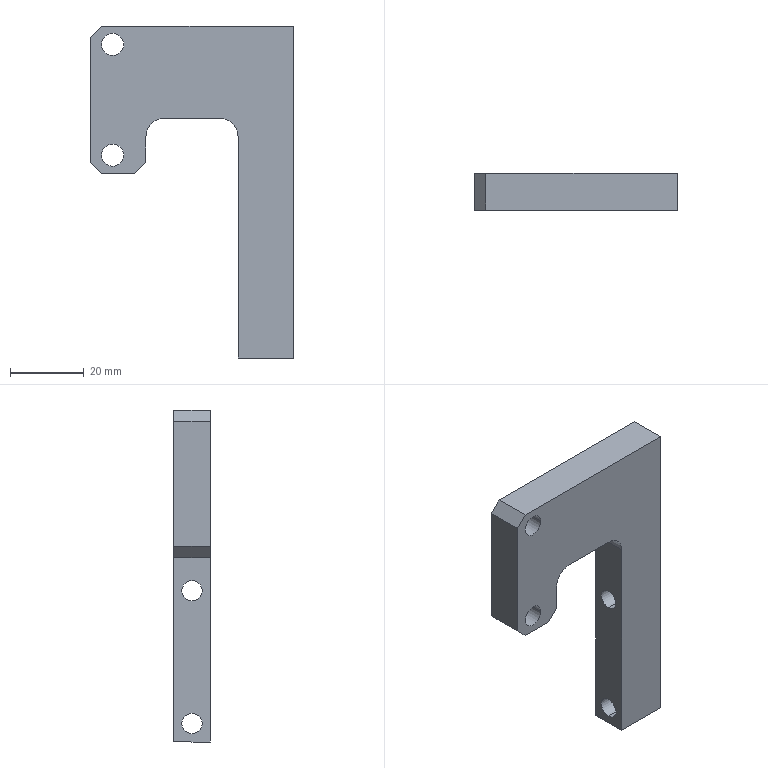Component | SolidWorks | JL001-05-01-011-1 | 1 solid | 23 faces | box 55 x 10 x 90 mm | volume 24444 mm3 | plane 13 | cylinder 10 | commonest cylinder face diameters 6 x4 5.5 x4 10 x2
build123d program:
from build123d import *

# Parameters (mm, degrees)
SKETCH1_W                  = 90
SKETCH1_H                  = 55
BOSS_EXTRUDE1_DEPTH        = 5
SKETCH2_W                  = 50
SKETCH2_H                  = 40
CUT_EXTRUDE1_DEPTH         = 54.677
SKETCH7_W                  = 15
SKETCH7_H                  = 25
CUT_EXTRUDE2_DEPTH         = 10
FILLET1_R                  = 5
F_5_5_5_5_DIAMETER_HOLE1_D = 5.5
M6_TAPPED_HOLE1_D          = 6
CHAMFER1_SIZE              = 3


with BuildPart() as part:
    # Sketch1 → Boss-Extrude1 (new, symmetric)
    with BuildSketch(Plane(origin=(0, 0, 0), x_dir=(1, 0, 0), z_dir=(0, 1, 0))):
        Rectangle(SKETCH1_W, SKETCH1_H)
    extrude(amount=BOSS_EXTRUDE1_DEPTH, both=True)

    # Sketch2 → Cut-Extrude1 (cut, through all)
    with BuildSketch(Plane(origin=(0, 5, 0), x_dir=(1, 0, 0), z_dir=(0, 1, 0))):
        with Locations((-20, -7.5)):
            Rectangle(SKETCH2_W, SKETCH2_H)
    extrude(amount=-CUT_EXTRUDE1_DEPTH, mode=Mode.SUBTRACT)

    # Sketch7 → Cut-Extrude2 (cut)
    with BuildSketch(Plane(origin=(0, 5, 0), x_dir=(1, 0, 0), z_dir=(0, 1, 0))):
        with Locations((12.5, 0)):
            Rectangle(SKETCH7_W, SKETCH7_H)
    extrude(amount=-CUT_EXTRUDE2_DEPTH, mode=Mode.SUBTRACT)

    # Fillet1
    fillet1_edges = [part.edges().sort_by_distance(p)[0] for p in [
        (20, 0, -12.5),
        (20, 0, 12.5),
    ]]
    fillet(fillet1_edges, radius=FILLET1_R)

    # 5.5 _5.5_ Diameter Hole1 (through all)
    with Locations(Plane.XY.offset(-12.5)):
        with Locations((-40, 0), (-4, 0)):
            Hole(F_5_5_5_5_DIAMETER_HOLE1_D / 2)

    # M6 Tapped Hole1 (through all)
    with Locations(Plane(origin=(0, 5, 0), x_dir=(1, 0, 0), z_dir=(0, 1, 0))):
        with Locations((10, -21.5), (40, -21.5)):
            Hole(M6_TAPPED_HOLE1_D / 2)

    # Chamfer1
    chamfer1_edges = [part.edges().sort_by_distance(p)[0] for p in [
        (5, 0, 27.5),
        (5, 0, 12.5),
        (45, 0, 27.5),
    ]]
    chamfer(chamfer1_edges, length=CHAMFER1_SIZE)


solid = part.part

# Placed as in the assembly
solid = solid.moved(Location((-47.5, 1130, 25), (0, -90, 0)))
STEP:
#1=COLOUR_RGB('',0.7922,0.8196,0.9333);
#2=FILL_AREA_STYLE_COLOUR('',#1);
#3=FILL_AREA_STYLE('',(#2));
#4=SURFACE_STYLE_FILL_AREA(#3);
#5=SURFACE_SIDE_STYLE('',(#4));
#6=SURFACE_STYLE_USAGE(.BOTH.,#5);
#7=PRESENTATION_STYLE_ASSIGNMENT((#6));
#8=CARTESIAN_POINT('',(-2.598,44.291,2.559));
#9=VERTEX_POINT('',#8);
#10=CARTESIAN_POINT('',(-2.835,44.291,2.559));
#11=VERTEX_POINT('',#10);
#12=CARTESIAN_POINT('',(-2.717,44.291,2.559));
#13=DIRECTION('',(-0.,1.,0.));
#14=DIRECTION('',(-1.,0.,0.));
#15=AXIS2_PLACEMENT_3D('',#12,#13,#14);
#16=CIRCLE('',#15,0.1181);
#17=EDGE_CURVE('',#9,#11,#16,.T.);
#18=ORIENTED_EDGE('',*,*,#17,.F.);
#19=CARTESIAN_POINT('',(-2.598,44.685,2.559));
#20=VERTEX_POINT('',#19);
#21=CARTESIAN_POINT('',(-2.598,44.685,2.559));
#22=DIRECTION('',(-0.,1.,0.));
#23=VECTOR('',#22,39.37);
#24=LINE('',#21,#23);
#25=EDGE_CURVE('',#9,#20,#24,.T.);
#26=ORIENTED_EDGE('',*,*,#25,.T.);
#27=CARTESIAN_POINT('',(-2.835,44.685,2.559));
#28=VERTEX_POINT('',#27);
#29=CARTESIAN_POINT('',(-2.717,44.685,2.559));
#30=DIRECTION('',(-0.,1.,0.));
#31=DIRECTION('',(-1.,0.,0.));
#32=AXIS2_PLACEMENT_3D('',#29,#30,#31);
#33=CIRCLE('',#32,0.1181);
#34=EDGE_CURVE('',#20,#28,#33,.T.);
#35=ORIENTED_EDGE('',*,*,#34,.T.);
#36=CARTESIAN_POINT('',(-2.835,44.685,2.559));
#37=DIRECTION('',(-0.,1.,0.));
#38=VECTOR('',#37,39.37);
#39=LINE('',#36,#38);
#40=EDGE_CURVE('',#11,#28,#39,.T.);
#41=ORIENTED_EDGE('',*,*,#40,.F.);
#42=EDGE_LOOP('',(#18,#26,#35,#41));
#43=FACE_OUTER_BOUND('',#42,.T.);
#44=CARTESIAN_POINT('',(-2.717,44.685,2.559));
#45=DIRECTION('',(-0.,1.,0.));
#46=DIRECTION('',(-1.,0.,0.));
#47=AXIS2_PLACEMENT_3D('',#44,#45,#46);
#48=CYLINDRICAL_SURFACE('',#47,0.1181);
#49=ADVANCED_FACE('',(#43),#48,.F.);
#50=CARTESIAN_POINT('',(-2.598,44.291,1.378));
#51=VERTEX_POINT('',#50);
#52=CARTESIAN_POINT('',(-2.835,44.291,1.378));
#53=VERTEX_POINT('',#52);
#54=CARTESIAN_POINT('',(-2.717,44.291,1.378));
#55=DIRECTION('',(-0.,1.,0.));
#56=DIRECTION('',(-1.,0.,0.));
#57=AXIS2_PLACEMENT_3D('',#54,#55,#56);
#58=CIRCLE('',#57,0.1181);
#59=EDGE_CURVE('',#51,#53,#58,.T.);
#60=ORIENTED_EDGE('',*,*,#59,.F.);
#61=CARTESIAN_POINT('',(-2.598,44.685,1.378));
#62=VERTEX_POINT('',#61);
#63=CARTESIAN_POINT('',(-2.598,44.685,1.378));
#64=DIRECTION('',(-0.,1.,0.));
#65=VECTOR('',#64,39.37);
#66=LINE('',#63,#65);
#67=EDGE_CURVE('',#51,#62,#66,.T.);
#68=ORIENTED_EDGE('',*,*,#67,.T.);
#69=CARTESIAN_POINT('',(-2.835,44.685,1.378));
#70=VERTEX_POINT('',#69);
#71=CARTESIAN_POINT('',(-2.717,44.685,1.378));
#72=DIRECTION('',(-0.,1.,0.));
#73=DIRECTION('',(-1.,0.,0.));
#74=AXIS2_PLACEMENT_3D('',#71,#72,#73);
#75=CIRCLE('',#74,0.1181);
#76=EDGE_CURVE('',#62,#70,#75,.T.);
#77=ORIENTED_EDGE('',*,*,#76,.T.);
#78=CARTESIAN_POINT('',(-2.835,44.685,1.378));
#79=DIRECTION('',(-0.,1.,0.));
#80=VECTOR('',#79,39.37);
#81=LINE('',#78,#80);
#82=EDGE_CURVE('',#53,#70,#81,.T.);
#83=ORIENTED_EDGE('',*,*,#82,.F.);
#84=EDGE_LOOP('',(#60,#68,#77,#83));
#85=FACE_OUTER_BOUND('',#84,.T.);
#86=CARTESIAN_POINT('',(-2.717,44.685,1.378));
#87=DIRECTION('',(-0.,1.,0.));
#88=DIRECTION('',(-1.,0.,0.));
#89=AXIS2_PLACEMENT_3D('',#86,#87,#88);
#90=CYLINDRICAL_SURFACE('',#89,0.1181);
#91=ADVANCED_FACE('',(#85),#90,.F.);
#92=CARTESIAN_POINT('',(-0.7874,44.488,-0.6988));
#93=VERTEX_POINT('',#92);
#94=CARTESIAN_POINT('',(-0.7874,44.488,-0.4823));
#95=VERTEX_POINT('',#94);
#96=CARTESIAN_POINT('',(-0.7874,44.488,-0.5906));
#97=DIRECTION('',(-1.,-0.,0.));
#98=DIRECTION('',(0.,0.,1.));
#99=AXIS2_PLACEMENT_3D('',#96,#97,#98);
#100=CIRCLE('',#99,0.1083);
#101=EDGE_CURVE('',#93,#95,#100,.T.);
#102=ORIENTED_EDGE('',*,*,#101,.F.);
#103=CARTESIAN_POINT('',(-1.378,44.488,-0.6988));
#104=VERTEX_POINT('',#103);
#105=CARTESIAN_POINT('',(-1.378,44.488,-0.6988));
#106=DIRECTION('',(-1.,-0.,0.));
#107=VECTOR('',#106,39.37);
#108=LINE('',#105,#107);
#109=EDGE_CURVE('',#93,#104,#108,.T.);
#110=ORIENTED_EDGE('',*,*,#109,.T.);
#111=CARTESIAN_POINT('',(-1.378,44.488,-0.4823));
#112=VERTEX_POINT('',#111);
#113=CARTESIAN_POINT('',(-1.378,44.488,-0.5906));
#114=DIRECTION('',(-1.,-0.,0.));
#115=DIRECTION('',(0.,0.,1.));
#116=AXIS2_PLACEMENT_3D('',#113,#114,#115);
#117=CIRCLE('',#116,0.1083);
#118=EDGE_CURVE('',#104,#112,#117,.T.);
#119=ORIENTED_EDGE('',*,*,#118,.T.);
#120=CARTESIAN_POINT('',(-1.378,44.488,-0.4823));
#121=DIRECTION('',(-1.,-0.,0.));
#122=VECTOR('',#121,39.37);
#123=LINE('',#120,#122);
#124=EDGE_CURVE('',#95,#112,#123,.T.);
#125=ORIENTED_EDGE('',*,*,#124,.F.);
#126=EDGE_LOOP('',(#102,#110,#119,#125));
#127=FACE_OUTER_BOUND('',#126,.T.);
#128=CARTESIAN_POINT('',(-1.378,44.488,-0.5906));
#129=DIRECTION('',(-1.,-0.,0.));
#130=DIRECTION('',(0.,0.,1.));
#131=AXIS2_PLACEMENT_3D('',#128,#129,#130);
#132=CYLINDRICAL_SURFACE('',#131,0.1083);
#133=ADVANCED_FACE('',(#127),#132,.F.);
#134=CARTESIAN_POINT('',(-0.7874,44.488,0.7185));
#135=VERTEX_POINT('',#134);
#136=CARTESIAN_POINT('',(-0.7874,44.488,0.935));
#137=VERTEX_POINT('',#136);
#138=CARTESIAN_POINT('',(-0.7874,44.488,0.8268));
#139=DIRECTION('',(-1.,-0.,0.));
#140=DIRECTION('',(0.,0.,1.));
#141=AXIS2_PLACEMENT_3D('',#138,#139,#140);
#142=CIRCLE('',#141,0.1083);
#143=EDGE_CURVE('',#135,#137,#142,.T.);
#144=ORIENTED_EDGE('',*,*,#143,.F.);
#145=CARTESIAN_POINT('',(-1.378,44.488,0.7185));
#146=VERTEX_POINT('',#145);
#147=CARTESIAN_POINT('',(-1.378,44.488,0.7185));
#148=DIRECTION('',(-1.,-0.,0.));
#149=VECTOR('',#148,39.37);
#150=LINE('',#147,#149);
#151=EDGE_CURVE('',#135,#146,#150,.T.);
#152=ORIENTED_EDGE('',*,*,#151,.T.);
#153=CARTESIAN_POINT('',(-1.378,44.488,0.935));
#154=VERTEX_POINT('',#153);
#155=CARTESIAN_POINT('',(-1.378,44.488,0.8268));
#156=DIRECTION('',(-1.,-0.,0.));
#157=DIRECTION('',(0.,0.,1.));
#158=AXIS2_PLACEMENT_3D('',#155,#156,#157);
#159=CIRCLE('',#158,0.1083);
#160=EDGE_CURVE('',#146,#154,#159,.T.);
#161=ORIENTED_EDGE('',*,*,#160,.T.);
#162=CARTESIAN_POINT('',(-1.378,44.488,0.935));
#163=DIRECTION('',(-1.,-0.,0.));
#164=VECTOR('',#163,39.37);
#165=LINE('',#162,#164);
#166=EDGE_CURVE('',#137,#154,#165,.T.);
#167=ORIENTED_EDGE('',*,*,#166,.F.);
#168=EDGE_LOOP('',(#144,#152,#161,#167));
#169=FACE_OUTER_BOUND('',#168,.T.);
#170=CARTESIAN_POINT('',(-1.378,44.488,0.8268));
#171=DIRECTION('',(-1.,-0.,0.));
#172=DIRECTION('',(0.,0.,1.));
#173=AXIS2_PLACEMENT_3D('',#170,#171,#172);
#174=CYLINDRICAL_SURFACE('',#173,0.1083);
#175=ADVANCED_FACE('',(#169),#174,.F.);
#176=CARTESIAN_POINT('',(-2.835,44.685,2.756));
#177=VERTEX_POINT('',#176);
#178=CARTESIAN_POINT('',(-0.7874,44.685,2.756));
#179=VERTEX_POINT('',#178);
#180=CARTESIAN_POINT('',(-0.7874,44.685,2.756));
#181=DIRECTION('',(1.,0.,-0.));
#182=VECTOR('',#181,39.37);
#183=LINE('',#180,#182);
#184=EDGE_CURVE('',#177,#179,#183,.T.);
#185=ORIENTED_EDGE('',*,*,#184,.F.);
#186=CARTESIAN_POINT('',(-2.835,44.291,2.756));
#187=VERTEX_POINT('',#186);
#188=CARTESIAN_POINT('',(-2.835,44.685,2.756));
#189=DIRECTION('',(0.,-1.,-0.));
#190=VECTOR('',#189,39.37);
#191=LINE('',#188,#190);
#192=EDGE_CURVE('',#177,#187,#191,.T.);
#193=ORIENTED_EDGE('',*,*,#192,.T.);
#194=CARTESIAN_POINT('',(-0.7874,44.291,2.756));
#195=VERTEX_POINT('',#194);
#196=CARTESIAN_POINT('',(-0.7874,44.291,2.756));
#197=DIRECTION('',(1.,0.,-0.));
#198=VECTOR('',#197,39.37);
#199=LINE('',#196,#198);
#200=EDGE_CURVE('',#187,#195,#199,.T.);
#201=ORIENTED_EDGE('',*,*,#200,.T.);
#202=CARTESIAN_POINT('',(-0.7874,44.685,2.756));
#203=DIRECTION('',(0.,-1.,-0.));
#204=VECTOR('',#203,39.37);
#205=LINE('',#202,#204);
#206=EDGE_CURVE('',#179,#195,#205,.T.);
#207=ORIENTED_EDGE('',*,*,#206,.F.);
#208=EDGE_LOOP('',(#185,#193,#201,#207));
#209=FACE_OUTER_BOUND('',#208,.T.);
#210=CARTESIAN_POINT('',(-0.7874,44.685,2.756));
#211=DIRECTION('',(-0.,0.,-1.));
#212=DIRECTION('',(-1.,-0.,0.));
#213=AXIS2_PLACEMENT_3D('',#210,#211,#212);
#214=PLANE('',#213);
#215=ADVANCED_FACE('',(#209),#214,.F.);
#216=CARTESIAN_POINT('',(-0.7874,44.488,-0.5906));
#217=DIRECTION('',(-1.,-0.,0.));
#218=DIRECTION('',(0.,0.,1.));
#219=AXIS2_PLACEMENT_3D('',#216,#217,#218);
#220=CIRCLE('',#219,0.1083);
#221=EDGE_CURVE('',#95,#93,#220,.T.);
#222=ORIENTED_EDGE('',*,*,#221,.T.);
#223=ORIENTED_EDGE('',*,*,#101,.T.);
#224=EDGE_LOOP('',(#222,#223));
#225=FACE_BOUND('',#224,.T.);
#226=CARTESIAN_POINT('',(-0.7874,44.488,0.8268));
#227=DIRECTION('',(-1.,-0.,0.));
#228=DIRECTION('',(0.,0.,1.));
#229=AXIS2_PLACEMENT_3D('',#226,#227,#228);
#230=CIRCLE('',#229,0.1083);
#231=EDGE_CURVE('',#137,#135,#230,.T.);
#232=ORIENTED_EDGE('',*,*,#231,.T.);
#233=ORIENTED_EDGE('',*,*,#143,.T.);
#234=EDGE_LOOP('',(#232,#233));
#235=FACE_BOUND('',#234,.T.);
#236=CARTESIAN_POINT('',(-0.7874,44.291,-0.7874));
#237=VERTEX_POINT('',#236);
#238=CARTESIAN_POINT('',(-0.7874,44.291,-0.7874));
#239=DIRECTION('',(-0.,0.,-1.));
#240=VECTOR('',#239,39.37);
#241=LINE('',#238,#240);
#242=EDGE_CURVE('',#195,#237,#241,.T.);
#243=ORIENTED_EDGE('',*,*,#242,.T.);
#244=CARTESIAN_POINT('',(-0.7874,44.685,-0.7874));
#245=VERTEX_POINT('',#244);
#246=CARTESIAN_POINT('',(-0.7874,44.685,-0.7874));
#247=DIRECTION('',(0.,-1.,-0.));
#248=VECTOR('',#247,39.37);
#249=LINE('',#246,#248);
#250=EDGE_CURVE('',#245,#237,#249,.T.);
#251=ORIENTED_EDGE('',*,*,#250,.F.);
#252=CARTESIAN_POINT('',(-0.7874,44.685,-0.7874));
#253=DIRECTION('',(-0.,0.,-1.));
#254=VECTOR('',#253,39.37);
#255=LINE('',#252,#254);
#256=EDGE_CURVE('',#179,#245,#255,.T.);
#257=ORIENTED_EDGE('',*,*,#256,.F.);
#258=ORIENTED_EDGE('',*,*,#206,.T.);
#259=EDGE_LOOP('',(#243,#251,#257,#258));
#260=FACE_OUTER_BOUND('',#259,.T.);
#261=CARTESIAN_POINT('',(-0.7874,44.685,-0.7874));
#262=DIRECTION('',(-1.,-0.,0.));
#263=DIRECTION('',(0.,-0.,1.));
#264=AXIS2_PLACEMENT_3D('',#261,#262,#263);
#265=PLANE('',#264);
#266=ADVANCED_FACE('',(#225,#235,#260),#265,.F.);
#267=CARTESIAN_POINT('',(-1.378,44.291,-0.7874));
#268=VERTEX_POINT('',#267);
#269=CARTESIAN_POINT('',(-0.7874,44.291,-0.7874));
#270=DIRECTION('',(-1.,-0.,0.));
#271=VECTOR('',#270,39.37);
#272=LINE('',#269,#271);
#273=EDGE_CURVE('',#237,#268,#272,.T.);
#274=ORIENTED_EDGE('',*,*,#273,.T.);
#275=CARTESIAN_POINT('',(-1.378,44.685,-0.7874));
#276=VERTEX_POINT('',#275);
#277=CARTESIAN_POINT('',(-1.378,44.291,-0.7874));
#278=DIRECTION('',(-0.,1.,0.));
#279=VECTOR('',#278,39.37);
#280=LINE('',#277,#279);
#281=EDGE_CURVE('',#268,#276,#280,.T.);
#282=ORIENTED_EDGE('',*,*,#281,.T.);
#283=CARTESIAN_POINT('',(-0.7874,44.685,-0.7874));
#284=DIRECTION('',(-1.,-0.,0.));
#285=VECTOR('',#284,39.37);
#286=LINE('',#283,#285);
#287=EDGE_CURVE('',#245,#276,#286,.T.);
#288=ORIENTED_EDGE('',*,*,#287,.F.);
#289=ORIENTED_EDGE('',*,*,#250,.T.);
#290=EDGE_LOOP('',(#274,#282,#288,#289));
#291=FACE_OUTER_BOUND('',#290,.T.);
#292=CARTESIAN_POINT('',(-0.7874,44.685,-0.7874));
#293=DIRECTION('',(0.,-0.,1.));
#294=DIRECTION('',(1.,0.,-0.));
#295=AXIS2_PLACEMENT_3D('',#292,#293,#294);
#296=PLANE('',#295);
#297=ADVANCED_FACE('',(#291),#296,.F.);
#298=CARTESIAN_POINT('',(-2.953,44.685,1.299));
#299=VERTEX_POINT('',#298);
#300=CARTESIAN_POINT('',(-2.953,44.685,2.638));
#301=VERTEX_POINT('',#300);
#302=CARTESIAN_POINT('',(-2.953,44.685,-0.7874));
#303=DIRECTION('',(0.,-0.,1.));
#304=VECTOR('',#303,39.37);
#305=LINE('',#302,#304);
#306=EDGE_CURVE('',#299,#301,#305,.T.);
#307=ORIENTED_EDGE('',*,*,#306,.F.);
#308=CARTESIAN_POINT('',(-2.953,44.291,1.299));
#309=VERTEX_POINT('',#308);
#310=CARTESIAN_POINT('',(-2.953,44.685,1.299));
#311=DIRECTION('',(0.,-1.,-0.));
#312=VECTOR('',#311,39.37);
#313=LINE('',#310,#312);
#314=EDGE_CURVE('',#299,#309,#313,.T.);
#315=ORIENTED_EDGE('',*,*,#314,.T.);
#316=CARTESIAN_POINT('',(-2.953,44.291,2.638));
#317=VERTEX_POINT('',#316);
#318=CARTESIAN_POINT('',(-2.953,44.291,-0.7874));
#319=DIRECTION('',(0.,-0.,1.));
#320=VECTOR('',#319,39.37);
#321=LINE('',#318,#320);
#322=EDGE_CURVE('',#309,#317,#321,.T.);
#323=ORIENTED_EDGE('',*,*,#322,.T.);
#324=CARTESIAN_POINT('',(-2.953,44.685,2.638));
#325=DIRECTION('',(-0.,1.,0.));
#326=VECTOR('',#325,39.37);
#327=LINE('',#324,#326);
#328=EDGE_CURVE('',#317,#301,#327,.T.);
#329=ORIENTED_EDGE('',*,*,#328,.T.);
#330=EDGE_LOOP('',(#307,#315,#323,#329));
#331=FACE_OUTER_BOUND('',#330,.T.);
#332=CARTESIAN_POINT('',(-2.953,44.685,-0.7874));
#333=DIRECTION('',(1.,0.,-0.));
#334=DIRECTION('',(-0.,0.,-1.));
#335=AXIS2_PLACEMENT_3D('',#332,#333,#334);
#336=PLANE('',#335);
#337=ADVANCED_FACE('',(#331),#336,.F.);
#338=CARTESIAN_POINT('',(-2.717,44.685,2.559));
#339=DIRECTION('',(-0.,1.,0.));
#340=DIRECTION('',(-1.,0.,0.));
#341=AXIS2_PLACEMENT_3D('',#338,#339,#340);
#342=CIRCLE('',#341,0.1181);
#343=EDGE_CURVE('',#28,#20,#342,.T.);
#344=ORIENTED_EDGE('',*,*,#343,.F.);
#345=ORIENTED_EDGE('',*,*,#34,.F.);
#346=EDGE_LOOP('',(#344,#345));
#347=FACE_BOUND('',#346,.T.);
#348=CARTESIAN_POINT('',(-2.717,44.685,1.378));
#349=DIRECTION('',(-0.,1.,0.));
#350=DIRECTION('',(-1.,0.,0.));
#351=AXIS2_PLACEMENT_3D('',#348,#349,#350);
#352=CIRCLE('',#351,0.1181);
#353=EDGE_CURVE('',#70,#62,#352,.T.);
#354=ORIENTED_EDGE('',*,*,#353,.F.);
#355=ORIENTED_EDGE('',*,*,#76,.F.);
#356=EDGE_LOOP('',(#354,#355));
#357=FACE_BOUND('',#356,.T.);
#358=CARTESIAN_POINT('',(-2.362,44.685,1.299));
#359=VERTEX_POINT('',#358);
#360=CARTESIAN_POINT('',(-2.362,44.685,1.575));
#361=VERTEX_POINT('',#360);
#362=CARTESIAN_POINT('',(-2.362,44.685,1.181));
#363=DIRECTION('',(0.,-0.,1.));
#364=VECTOR('',#363,39.37);
#365=LINE('',#362,#364);
#366=EDGE_CURVE('',#359,#361,#365,.T.);
#367=ORIENTED_EDGE('',*,*,#366,.F.);
#368=CARTESIAN_POINT('',(-2.48,44.685,1.181));
#369=VERTEX_POINT('',#368);
#370=CARTESIAN_POINT('',(-2.274,44.685,1.388));
#371=DIRECTION('',(-0.7071,0.,-0.7071));
#372=VECTOR('',#371,39.37);
#373=LINE('',#370,#372);
#374=EDGE_CURVE('',#359,#369,#373,.T.);
#375=ORIENTED_EDGE('',*,*,#374,.T.);
#376=CARTESIAN_POINT('',(-2.835,44.685,1.181));
#377=VERTEX_POINT('',#376);
#378=CARTESIAN_POINT('',(-1.378,44.685,1.181));
#379=DIRECTION('',(1.,0.,-0.));
#380=VECTOR('',#379,39.37);
#381=LINE('',#378,#380);
#382=EDGE_CURVE('',#377,#369,#381,.T.);
#383=ORIENTED_EDGE('',*,*,#382,.F.);
#384=CARTESIAN_POINT('',(-2.254,44.685,0.6004));
#385=DIRECTION('',(-0.7071,-0.,0.7071));
#386=VECTOR('',#385,39.37);
#387=LINE('',#384,#386);
#388=EDGE_CURVE('',#377,#299,#387,.T.);
#389=ORIENTED_EDGE('',*,*,#388,.T.);
#390=ORIENTED_EDGE('',*,*,#306,.T.);
#391=CARTESIAN_POINT('',(-3.238,44.685,2.352));
#392=DIRECTION('',(0.7071,-0.,0.7071));
#393=VECTOR('',#392,39.37);
#394=LINE('',#391,#393);
#395=EDGE_CURVE('',#301,#177,#394,.T.);
#396=ORIENTED_EDGE('',*,*,#395,.T.);
#397=ORIENTED_EDGE('',*,*,#184,.T.);
#398=ORIENTED_EDGE('',*,*,#256,.T.);
#399=ORIENTED_EDGE('',*,*,#287,.T.);
#400=CARTESIAN_POINT('',(-1.378,44.685,1.575));
#401=VERTEX_POINT('',#400);
#402=CARTESIAN_POINT('',(-1.378,44.685,-0.7874));
#403=DIRECTION('',(-0.,0.,-1.));
#404=VECTOR('',#403,39.37);
#405=LINE('',#402,#404);
#406=EDGE_CURVE('',#401,#276,#405,.T.);
#407=ORIENTED_EDGE('',*,*,#406,.F.);
#408=CARTESIAN_POINT('',(-1.575,44.685,1.772));
#409=VERTEX_POINT('',#408);
#410=CARTESIAN_POINT('',(-1.575,44.685,1.575));
#411=DIRECTION('',(0.,-1.,-0.));
#412=DIRECTION('',(-1.,0.,0.));
#413=AXIS2_PLACEMENT_3D('',#410,#411,#412);
#414=CIRCLE('',#413,0.1969);
#415=EDGE_CURVE('',#401,#409,#414,.T.);
#416=ORIENTED_EDGE('',*,*,#415,.T.);
#417=CARTESIAN_POINT('',(-2.165,44.685,1.772));
#418=VERTEX_POINT('',#417);
#419=CARTESIAN_POINT('',(-1.378,44.685,1.772));
#420=DIRECTION('',(1.,0.,-0.));
#421=VECTOR('',#420,39.37);
#422=LINE('',#419,#421);
#423=EDGE_CURVE('',#418,#409,#422,.T.);
#424=ORIENTED_EDGE('',*,*,#423,.F.);
#425=CARTESIAN_POINT('',(-2.165,44.685,1.575));
#426=DIRECTION('',(0.,-1.,-0.));
#427=DIRECTION('',(-1.,0.,0.));
#428=AXIS2_PLACEMENT_3D('',#425,#426,#427);
#429=CIRCLE('',#428,0.1969);
#430=EDGE_CURVE('',#418,#361,#429,.T.);
#431=ORIENTED_EDGE('',*,*,#430,.T.);
#432=EDGE_LOOP('',(#367,#375,#383,#389,#390,#396,#397,#398,#399,#407,#416,#424,#431));
#433=FACE_OUTER_BOUND('',#432,.T.);
#434=CARTESIAN_POINT('',(-1.87,44.685,0.9843));
#435=DIRECTION('',(-0.,1.,0.));
#436=DIRECTION('',(-1.,-0.,0.));
#437=AXIS2_PLACEMENT_3D('',#434,#435,#436);
#438=PLANE('',#437);
#439=ADVANCED_FACE('',(#347,#357,#433),#438,.T.);
#440=CARTESIAN_POINT('',(-2.717,44.291,2.559));
#441=DIRECTION('',(-0.,1.,0.));
#442=DIRECTION('',(-1.,0.,0.));
#443=AXIS2_PLACEMENT_3D('',#440,#441,#442);
#444=CIRCLE('',#443,0.1181);
#445=EDGE_CURVE('',#11,#9,#444,.T.);
#446=ORIENTED_EDGE('',*,*,#445,.T.);
#447=ORIENTED_EDGE('',*,*,#17,.T.);
#448=EDGE_LOOP('',(#446,#447));
#449=FACE_BOUND('',#448,.T.);
#450=CARTESIAN_POINT('',(-2.717,44.291,1.378));
#451=DIRECTION('',(-0.,1.,0.));
#452=DIRECTION('',(-1.,0.,0.));
#453=AXIS2_PLACEMENT_3D('',#450,#451,#452);
#454=CIRCLE('',#453,0.1181);
#455=EDGE_CURVE('',#53,#51,#454,.T.);
#456=ORIENTED_EDGE('',*,*,#455,.T.);
#457=ORIENTED_EDGE('',*,*,#59,.T.);
#458=EDGE_LOOP('',(#456,#457));
#459=FACE_BOUND('',#458,.T.);
#460=CARTESIAN_POINT('',(-2.835,44.291,1.181));
#461=VERTEX_POINT('',#460);
#462=CARTESIAN_POINT('',(-2.48,44.291,1.181));
#463=VERTEX_POINT('',#462);
#464=CARTESIAN_POINT('',(-1.378,44.291,1.181));
#465=DIRECTION('',(1.,0.,-0.));
#466=VECTOR('',#465,39.37);
#467=LINE('',#464,#466);
#468=EDGE_CURVE('',#461,#463,#467,.T.);
#469=ORIENTED_EDGE('',*,*,#468,.T.);
#470=CARTESIAN_POINT('',(-2.362,44.291,1.299));
#471=VERTEX_POINT('',#470);
#472=CARTESIAN_POINT('',(-2.362,44.291,1.299));
#473=DIRECTION('',(0.7071,-0.,0.7071));
#474=VECTOR('',#473,39.37);
#475=LINE('',#472,#474);
#476=EDGE_CURVE('',#463,#471,#475,.T.);
#477=ORIENTED_EDGE('',*,*,#476,.T.);
#478=CARTESIAN_POINT('',(-2.362,44.291,1.575));
#479=VERTEX_POINT('',#478);
#480=CARTESIAN_POINT('',(-2.362,44.291,1.181));
#481=DIRECTION('',(0.,-0.,1.));
#482=VECTOR('',#481,39.37);
#483=LINE('',#480,#482);
#484=EDGE_CURVE('',#471,#479,#483,.T.);
#485=ORIENTED_EDGE('',*,*,#484,.T.);
#486=CARTESIAN_POINT('',(-2.165,44.291,1.772));
#487=VERTEX_POINT('',#486);
#488=CARTESIAN_POINT('',(-2.165,44.291,1.575));
#489=DIRECTION('',(-0.,1.,0.));
#490=DIRECTION('',(-1.,0.,0.));
#491=AXIS2_PLACEMENT_3D('',#488,#489,#490);
#492=CIRCLE('',#491,0.1969);
#493=EDGE_CURVE('',#479,#487,#492,.T.);
#494=ORIENTED_EDGE('',*,*,#493,.T.);
#495=CARTESIAN_POINT('',(-1.575,44.291,1.772));
#496=VERTEX_POINT('',#495);
#497=CARTESIAN_POINT('',(-1.378,44.291,1.772));
#498=DIRECTION('',(1.,0.,-0.));
#499=VECTOR('',#498,39.37);
#500=LINE('',#497,#499);
#501=EDGE_CURVE('',#487,#496,#500,.T.);
#502=ORIENTED_EDGE('',*,*,#501,.T.);
#503=CARTESIAN_POINT('',(-1.378,44.291,1.575));
#504=VERTEX_POINT('',#503);
#505=CARTESIAN_POINT('',(-1.575,44.291,1.575));
#506=DIRECTION('',(-0.,1.,0.));
#507=DIRECTION('',(-1.,0.,0.));
#508=AXIS2_PLACEMENT_3D('',#505,#506,#507);
#509=CIRCLE('',#508,0.1969);
#510=EDGE_CURVE('',#496,#504,#509,.T.);
#511=ORIENTED_EDGE('',*,*,#510,.T.);
#512=CARTESIAN_POINT('',(-1.378,44.291,-0.7874));
#513=DIRECTION('',(-0.,0.,-1.));
#514=VECTOR('',#513,39.37);
#515=LINE('',#512,#514);
#516=EDGE_CURVE('',#504,#268,#515,.T.);
#517=ORIENTED_EDGE('',*,*,#516,.T.);
#518=ORIENTED_EDGE('',*,*,#273,.F.);
#519=ORIENTED_EDGE('',*,*,#242,.F.);
#520=ORIENTED_EDGE('',*,*,#200,.F.);
#521=CARTESIAN_POINT('',(-2.835,44.291,2.756));
#522=DIRECTION('',(-0.7071,0.,-0.7071));
#523=VECTOR('',#522,39.37);
#524=LINE('',#521,#523);
#525=EDGE_CURVE('',#187,#317,#524,.T.);
#526=ORIENTED_EDGE('',*,*,#525,.T.);
#527=ORIENTED_EDGE('',*,*,#322,.F.);
#528=CARTESIAN_POINT('',(-2.835,44.291,1.181));
#529=DIRECTION('',(0.7071,0.,-0.7071));
#530=VECTOR('',#529,39.37);
#531=LINE('',#528,#530);
#532=EDGE_CURVE('',#309,#461,#531,.T.);
#533=ORIENTED_EDGE('',*,*,#532,.T.);
#534=EDGE_LOOP('',(#469,#477,#485,#494,#502,#511,#517,#518,#519,#520,#526,#527,#533));
#535=FACE_OUTER_BOUND('',#534,.T.);
#536=CARTESIAN_POINT('',(-1.87,44.291,0.9843));
#537=DIRECTION('',(-0.,1.,0.));
#538=DIRECTION('',(-1.,-0.,0.));
#539=AXIS2_PLACEMENT_3D('',#536,#537,#538);
#540=PLANE('',#539);
#541=ADVANCED_FACE('',(#449,#459,#535),#540,.F.);
#542=CARTESIAN_POINT('',(-1.378,44.488,-0.5906));
#543=DIRECTION('',(-1.,-0.,0.));
#544=DIRECTION('',(0.,0.,1.));
#545=AXIS2_PLACEMENT_3D('',#542,#543,#544);
#546=CIRCLE('',#545,0.1083);
#547=EDGE_CURVE('',#112,#104,#546,.T.);
#548=ORIENTED_EDGE('',*,*,#547,.F.);
#549=ORIENTED_EDGE('',*,*,#118,.F.);
#550=EDGE_LOOP('',(#548,#549));
#551=FACE_BOUND('',#550,.T.);
#552=CARTESIAN_POINT('',(-1.378,44.488,0.8268));
#553=DIRECTION('',(-1.,-0.,0.));
#554=DIRECTION('',(0.,0.,1.));
#555=AXIS2_PLACEMENT_3D('',#552,#553,#554);
#556=CIRCLE('',#555,0.1083);
#557=EDGE_CURVE('',#154,#146,#556,.T.);
#558=ORIENTED_EDGE('',*,*,#557,.F.);
#559=ORIENTED_EDGE('',*,*,#160,.F.);
#560=EDGE_LOOP('',(#558,#559));
#561=FACE_BOUND('',#560,.T.);
#562=ORIENTED_EDGE('',*,*,#516,.F.);
#563=CARTESIAN_POINT('',(-1.378,44.685,1.575));
#564=DIRECTION('',(-0.,1.,0.));
#565=VECTOR('',#564,39.37);
#566=LINE('',#563,#565);
#567=EDGE_CURVE('',#504,#401,#566,.T.);
#568=ORIENTED_EDGE('',*,*,#567,.T.);
#569=ORIENTED_EDGE('',*,*,#406,.T.);
#570=ORIENTED_EDGE('',*,*,#281,.F.);
#571=EDGE_LOOP('',(#562,#568,#569,#570));
#572=FACE_OUTER_BOUND('',#571,.T.);
#573=CARTESIAN_POINT('',(-1.378,44.291,-0.7874));
#574=DIRECTION('',(1.,0.,-0.));
#575=DIRECTION('',(-0.,0.,-1.));
#576=AXIS2_PLACEMENT_3D('',#573,#574,#575);
#577=PLANE('',#576);
#578=ADVANCED_FACE('',(#551,#561,#572),#577,.F.);
#579=ORIENTED_EDGE('',*,*,#382,.T.);
#580=CARTESIAN_POINT('',(-2.48,44.291,1.181));
#581=DIRECTION('',(0.,-1.,-0.));
#582=VECTOR('',#581,39.37);
#583=LINE('',#580,#582);
#584=EDGE_CURVE('',#369,#463,#583,.T.);
#585=ORIENTED_EDGE('',*,*,#584,.T.);
#586=ORIENTED_EDGE('',*,*,#468,.F.);
#587=CARTESIAN_POINT('',(-2.835,44.291,1.181));
#588=DIRECTION('',(-0.,1.,0.));
#589=VECTOR('',#588,39.37);
#590=LINE('',#587,#589);
#591=EDGE_CURVE('',#461,#377,#590,.T.);
#592=ORIENTED_EDGE('',*,*,#591,.T.);
#593=EDGE_LOOP('',(#579,#585,#586,#592));
#594=FACE_OUTER_BOUND('',#593,.T.);
#595=CARTESIAN_POINT('',(-1.378,44.291,1.181));
#596=DIRECTION('',(0.,-0.,1.));
#597=DIRECTION('',(1.,0.,-0.));
#598=AXIS2_PLACEMENT_3D('',#595,#596,#597);
#599=PLANE('',#598);
#600=ADVANCED_FACE('',(#594),#599,.F.);
#601=ORIENTED_EDGE('',*,*,#501,.F.);
#602=CARTESIAN_POINT('',(-2.165,44.685,1.772));
#603=DIRECTION('',(-0.,1.,0.));
#604=VECTOR('',#603,39.37);
#605=LINE('',#602,#604);
#606=EDGE_CURVE('',#487,#418,#605,.T.);
#607=ORIENTED_EDGE('',*,*,#606,.T.);
#608=ORIENTED_EDGE('',*,*,#423,.T.);
#609=CARTESIAN_POINT('',(-1.575,44.291,1.772));
#610=DIRECTION('',(0.,-1.,-0.));
#611=VECTOR('',#610,39.37);
#612=LINE('',#609,#611);
#613=EDGE_CURVE('',#409,#496,#612,.T.);
#614=ORIENTED_EDGE('',*,*,#613,.T.);
#615=EDGE_LOOP('',(#601,#607,#608,#614));
#616=FACE_OUTER_BOUND('',#615,.T.);
#617=CARTESIAN_POINT('',(-1.378,44.291,1.772));
#618=DIRECTION('',(0.,-0.,1.));
#619=DIRECTION('',(1.,0.,-0.));
#620=AXIS2_PLACEMENT_3D('',#617,#618,#619);
#621=PLANE('',#620);
#622=ADVANCED_FACE('',(#616),#621,.F.);
#623=ORIENTED_EDGE('',*,*,#484,.F.);
#624=CARTESIAN_POINT('',(-2.362,44.291,1.299));
#625=DIRECTION('',(-0.,1.,0.));
#626=VECTOR('',#625,39.37);
#627=LINE('',#624,#626);
#628=EDGE_CURVE('',#471,#359,#627,.T.);
#629=ORIENTED_EDGE('',*,*,#628,.T.);
#630=ORIENTED_EDGE('',*,*,#366,.T.);
#631=CARTESIAN_POINT('',(-2.362,44.291,1.575));
#632=DIRECTION('',(0.,-1.,-0.));
#633=VECTOR('',#632,39.37);
#634=LINE('',#631,#633);
#635=EDGE_CURVE('',#361,#479,#634,.T.);
#636=ORIENTED_EDGE('',*,*,#635,.T.);
#637=EDGE_LOOP('',(#623,#629,#630,#636));
#638=FACE_OUTER_BOUND('',#637,.T.);
#639=CARTESIAN_POINT('',(-2.362,44.291,1.181));
#640=DIRECTION('',(-1.,-0.,0.));
#641=DIRECTION('',(0.,-0.,1.));
#642=AXIS2_PLACEMENT_3D('',#639,#640,#641);
#643=PLANE('',#642);
#644=ADVANCED_FACE('',(#638),#643,.F.);
#645=ORIENTED_EDGE('',*,*,#493,.F.);
#646=ORIENTED_EDGE('',*,*,#635,.F.);
#647=ORIENTED_EDGE('',*,*,#430,.F.);
#648=ORIENTED_EDGE('',*,*,#606,.F.);
#649=EDGE_LOOP('',(#645,#646,#647,#648));
#650=FACE_OUTER_BOUND('',#649,.T.);
#651=CARTESIAN_POINT('',(-2.165,44.291,1.575));
#652=DIRECTION('',(0.,-1.,-0.));
#653=DIRECTION('',(1.,0.,0.));
#654=AXIS2_PLACEMENT_3D('',#651,#652,#653);
#655=CYLINDRICAL_SURFACE('',#654,0.1969);
#656=ADVANCED_FACE('',(#650),#655,.F.);
#657=ORIENTED_EDGE('',*,*,#510,.F.);
#658=ORIENTED_EDGE('',*,*,#613,.F.);
#659=ORIENTED_EDGE('',*,*,#415,.F.);
#660=ORIENTED_EDGE('',*,*,#567,.F.);
#661=EDGE_LOOP('',(#657,#658,#659,#660));
#662=FACE_OUTER_BOUND('',#661,.T.);
#663=CARTESIAN_POINT('',(-1.575,44.291,1.575));
#664=DIRECTION('',(0.,-1.,-0.));
#665=DIRECTION('',(1.,0.,0.));
#666=AXIS2_PLACEMENT_3D('',#663,#664,#665);
#667=CYLINDRICAL_SURFACE('',#666,0.1969);
#668=ADVANCED_FACE('',(#662),#667,.F.);
#669=ORIENTED_EDGE('',*,*,#151,.F.);
#670=ORIENTED_EDGE('',*,*,#231,.F.);
#671=ORIENTED_EDGE('',*,*,#166,.T.);
#672=ORIENTED_EDGE('',*,*,#557,.T.);
#673=EDGE_LOOP('',(#669,#670,#671,#672));
#674=FACE_OUTER_BOUND('',#673,.T.);
#675=CARTESIAN_POINT('',(-1.378,44.488,0.8268));
#676=DIRECTION('',(-1.,-0.,0.));
#677=DIRECTION('',(0.,0.,1.));
#678=AXIS2_PLACEMENT_3D('',#675,#676,#677);
#679=CYLINDRICAL_SURFACE('',#678,0.1083);
#680=ADVANCED_FACE('',(#674),#679,.F.);
#681=ORIENTED_EDGE('',*,*,#109,.F.);
#682=ORIENTED_EDGE('',*,*,#221,.F.);
#683=ORIENTED_EDGE('',*,*,#124,.T.);
#684=ORIENTED_EDGE('',*,*,#547,.T.);
#685=EDGE_LOOP('',(#681,#682,#683,#684));
#686=FACE_OUTER_BOUND('',#685,.T.);
#687=CARTESIAN_POINT('',(-1.378,44.488,-0.5906));
#688=DIRECTION('',(-1.,-0.,0.));
#689=DIRECTION('',(0.,0.,1.));
#690=AXIS2_PLACEMENT_3D('',#687,#688,#689);
#691=CYLINDRICAL_SURFACE('',#690,0.1083);
#692=ADVANCED_FACE('',(#686),#691,.F.);
#693=ORIENTED_EDGE('',*,*,#67,.F.);
#694=ORIENTED_EDGE('',*,*,#455,.F.);
#695=ORIENTED_EDGE('',*,*,#82,.T.);
#696=ORIENTED_EDGE('',*,*,#353,.T.);
#697=EDGE_LOOP('',(#693,#694,#695,#696));
#698=FACE_OUTER_BOUND('',#697,.T.);
#699=CARTESIAN_POINT('',(-2.717,44.685,1.378));
#700=DIRECTION('',(-0.,1.,0.));
#701=DIRECTION('',(-1.,0.,0.));
#702=AXIS2_PLACEMENT_3D('',#699,#700,#701);
#703=CYLINDRICAL_SURFACE('',#702,0.1181);
#704=ADVANCED_FACE('',(#698),#703,.F.);
#705=ORIENTED_EDGE('',*,*,#25,.F.);
#706=ORIENTED_EDGE('',*,*,#445,.F.);
#707=ORIENTED_EDGE('',*,*,#40,.T.);
#708=ORIENTED_EDGE('',*,*,#343,.T.);
#709=EDGE_LOOP('',(#705,#706,#707,#708));
#710=FACE_OUTER_BOUND('',#709,.T.);
#711=CARTESIAN_POINT('',(-2.717,44.685,2.559));
#712=DIRECTION('',(-0.,1.,0.));
#713=DIRECTION('',(-1.,0.,0.));
#714=AXIS2_PLACEMENT_3D('',#711,#712,#713);
#715=CYLINDRICAL_SURFACE('',#714,0.1181);
#716=ADVANCED_FACE('',(#710),#715,.F.);
#717=ORIENTED_EDGE('',*,*,#476,.F.);
#718=ORIENTED_EDGE('',*,*,#584,.F.);
#719=ORIENTED_EDGE('',*,*,#374,.F.);
#720=ORIENTED_EDGE('',*,*,#628,.F.);
#721=EDGE_LOOP('',(#717,#718,#719,#720));
#722=FACE_OUTER_BOUND('',#721,.T.);
#723=CARTESIAN_POINT('',(-2.362,44.291,1.299));
#724=DIRECTION('',(-0.7071,-0.,0.7071));
#725=DIRECTION('',(-0.,1.,0.));
#726=AXIS2_PLACEMENT_3D('',#723,#724,#725);
#727=PLANE('',#726);
#728=ADVANCED_FACE('',(#722),#727,.F.);
#729=ORIENTED_EDGE('',*,*,#532,.F.);
#730=ORIENTED_EDGE('',*,*,#314,.F.);
#731=ORIENTED_EDGE('',*,*,#388,.F.);
#732=ORIENTED_EDGE('',*,*,#591,.F.);
#733=EDGE_LOOP('',(#729,#730,#731,#732));
#734=FACE_OUTER_BOUND('',#733,.T.);
#735=CARTESIAN_POINT('',(-2.835,44.291,1.181));
#736=DIRECTION('',(0.7071,-0.,0.7071));
#737=DIRECTION('',(-0.,1.,0.));
#738=AXIS2_PLACEMENT_3D('',#735,#736,#737);
#739=PLANE('',#738);
#740=ADVANCED_FACE('',(#734),#739,.F.);
#741=ORIENTED_EDGE('',*,*,#395,.F.);
#742=ORIENTED_EDGE('',*,*,#328,.F.);
#743=ORIENTED_EDGE('',*,*,#525,.F.);
#744=ORIENTED_EDGE('',*,*,#192,.F.);
#745=EDGE_LOOP('',(#741,#742,#743,#744));
#746=FACE_OUTER_BOUND('',#745,.T.);
#747=CARTESIAN_POINT('',(-2.835,44.685,2.756));
#748=DIRECTION('',(0.7071,0.,-0.7071));
#749=DIRECTION('',(0.,-1.,-0.));
#750=AXIS2_PLACEMENT_3D('',#747,#748,#749);
#751=PLANE('',#750);
#752=ADVANCED_FACE('',(#746),#751,.F.);
#753=CLOSED_SHELL('',(#49,#91,#133,#175,#215,#266,#297,#337,#439,#541,#578,#600,#622,#644,#656,#668,#680,#692,#704,#716,#728,#740,#752));
#754=MANIFOLD_SOLID_BREP('',#753);
#755=STYLED_ITEM('',(#7),#754);
#756=PRESENTATION_LAYER_ASSIGNMENT('','',(#755));
#757=(LENGTH_UNIT()NAMED_UNIT(*)SI_UNIT($,.METRE.));
#758=LENGTH_MEASURE_WITH_UNIT(LENGTH_MEASURE(0.0254),#757);
#759=DIMENSIONAL_EXPONENTS(1.,0.,0.,0.,0.,0.,0.);
#760=(CONVERSION_BASED_UNIT('',#758)LENGTH_UNIT()NAMED_UNIT(#759));
#761=UNCERTAINTY_MEASURE_WITH_UNIT(LENGTH_MEASURE(0.00001),#760,'','');
#762=(NAMED_UNIT(*)PLANE_ANGLE_UNIT()SI_UNIT($,.RADIAN.));
#763=(NAMED_UNIT(*)SI_UNIT($,.STERADIAN.)SOLID_ANGLE_UNIT());
#764=(GEOMETRIC_REPRESENTATION_CONTEXT(3)GLOBAL_UNCERTAINTY_ASSIGNED_CONTEXT((#761))GLOBAL_UNIT_ASSIGNED_CONTEXT((#760,#762,#763))REPRESENTATION_CONTEXT('',''));
#765=MECHANICAL_DESIGN_GEOMETRIC_PRESENTATION_REPRESENTATION('',(#755),#764);
#766=CARTESIAN_POINT('',(0.,0.,0.));
#767=DIRECTION('',(0.,0.,1.));
#768=DIRECTION('',(1.,0.,0.));
#769=AXIS2_PLACEMENT_3D('',#766,#767,#768);
#770=(LENGTH_UNIT()NAMED_UNIT(*)SI_UNIT($,.METRE.));
#771=LENGTH_MEASURE_WITH_UNIT(LENGTH_MEASURE(0.0254),#770);
#772=DIMENSIONAL_EXPONENTS(1.,0.,0.,0.,0.,0.,0.);
#773=(CONVERSION_BASED_UNIT('',#771)LENGTH_UNIT()NAMED_UNIT(#772));
#774=UNCERTAINTY_MEASURE_WITH_UNIT(LENGTH_MEASURE(0.00001),#773,'','');
#775=(NAMED_UNIT(*)PLANE_ANGLE_UNIT()SI_UNIT($,.RADIAN.));
#776=(NAMED_UNIT(*)SI_UNIT($,.STERADIAN.)SOLID_ANGLE_UNIT());
#777=(GEOMETRIC_REPRESENTATION_CONTEXT(3)GLOBAL_UNCERTAINTY_ASSIGNED_CONTEXT((#774))GLOBAL_UNIT_ASSIGNED_CONTEXT((#773,#775,#776))REPRESENTATION_CONTEXT('',''));
#778=ADVANCED_BREP_SHAPE_REPRESENTATION('',(#754,#769),#777);